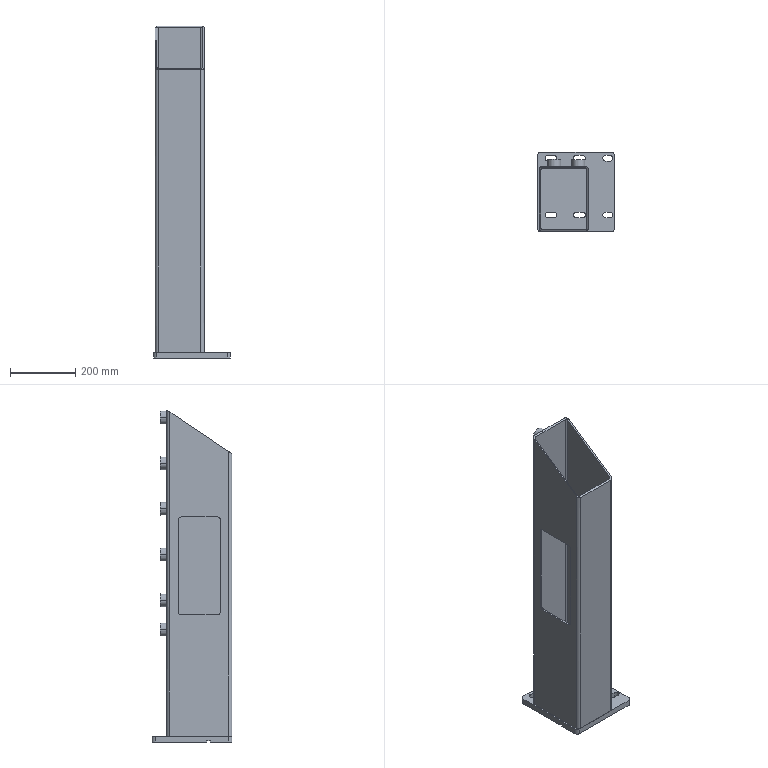Component | SolidWorks | 12ATransverseStraighteningSeat-1 | 8 solids | 129 faces | volume 3995935 mm3 | cylinder 72 | plane 57 | commonest cylinder face diameters 10.2 x24 18 x18 20 x14 40 x12 10 x4 | material Q235